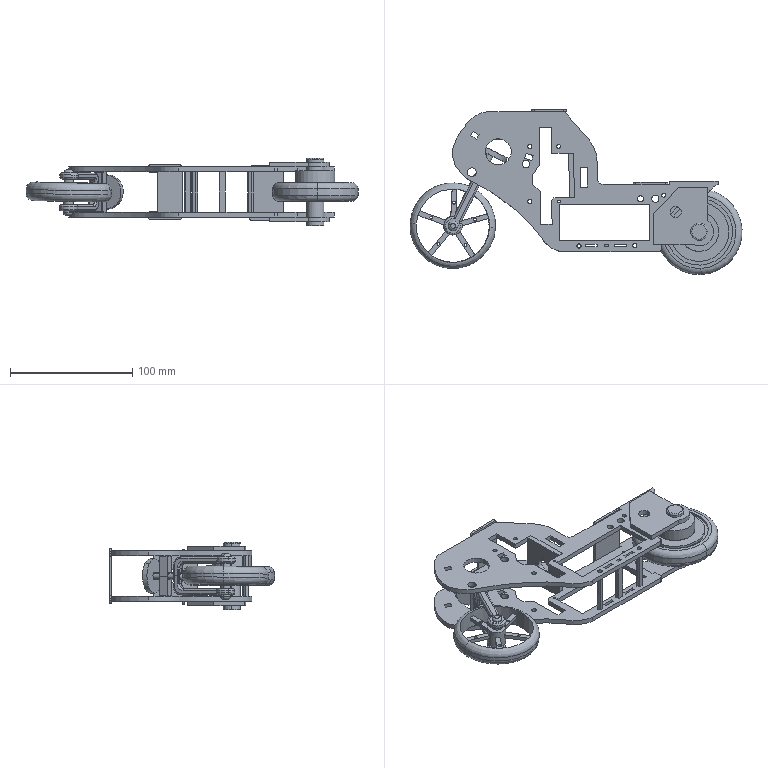Assembly | SolidWorks | mm | 17 component files | 18 solids | 481 faces | box 271.57 x 135.08 x 55 mm | volume 177248 mm3 | plane 239 | cylinder 194 | torus 36 | sphere 8 | spline 4 | commonest cylinder face diameters 2 x16 3 x13 1 x13 8 x10 2.368 x10 4 x10 15 x8 3.467 x8
Bill of materials:
ConnectingBlock1 | 1 |  | Elongated prismatic block, roughly square in cross-section, with lightly rounded edges and a single round cross hole through the side faces.
ConnectingBlock | 1 |  | U-shaped yoke/clevis-like bracket: two parallel arms joined by a rounded base, each arm ending in a flat ring eye with a round hole, and a round hole through the base web.
HexStandoff | 2 |  | Long hollow hexagonal-section tube with a circular bore running the full length; looks like a hex standoff or spacer.
LowerBaffle | 1 |  | Thin flat rectangular plate with rounded corners and four small round holes, one near each corner.
MiddleBaffle | 1 |  | Square flat plate with sharp edges, a large central circular through hole, and four small holes evenly spaced at 90 degrees on a circle around it.
MiddleShortPlate | 1 |  | Plain solid rectangular bar/prism with sharp edges and no holes or other features.
MirrorRearSidePlate1 | 1 |  | Flat plate with one chamfered (angled) corner, a smaller round hole, and a larger round hole set in a rounded lobe that sticks out past one edge.
MirrorSidePlate | 1 |  | Thin flat plate with a complex irregular outline (curved lobe on one end, long narrow tab on the other ending in a concave arc notch) and many cutouts: a large round hole, several small round holes, small rectangular slots, a cross-shaped opening, and a large rectangular window.
Motor | 1 |  | Stepped cylindrical pin with a wider disc-shaped collar near one end, a short cylindrical stub above the collar, and a longer shank of the same diameter below it; ends have small edge rounds.
Part15 | 1 |  | Flat circular disc with a single slender cylindrical pin sticking out perpendicular from the center of one face; pin tip is rounded or chamfered.
RearSidePlate1 | 1 |  | Flat plate with one chamfered (angled) corner, a smaller round hole, and a larger round hole set in a rounded lobe that sticks out past one edge.
RearWheel | 1 |  | Annular disc/ring with a well-rounded outer edge, a central through bore with a larger counterbore step on one face, and a shallow circular groove on that same face.
SidePlate | 1 |  | Thin flat plate with an irregular profile. One end is a rounded lobe and the other is a long narrow arm. The plate has a large round hole, several small round holes, small square/rectangular holes, a large rectangular window, a stepped cross-shaped cutout and a row of small slots.
Tire | 1 |  | Wheel-like ring with five spokes. It has an outer rim with a rounded (toroidal-looking) profile, an open center, and five straight flat spokes running from a cylindrical central hub with a round bore. Each spoke has one small through-hole.
UpperBaffle | 1 |  | Flat rectangular plate with rounded corners. One long side has a wide rectangular recess, which leaves two tabs. There are four small round through-holes, one near each corner, two of them in the tabs.
VehicleRearAxis | 1 |  | Solid round rod or pin with rounded or chamfered ends at both sides. The end view shows a circular cross-section with a slightly domed, faceted end face.
Mates:
1. concentric | Tire-1 face at (-9.114, -6.81, -21.475) dir (0.01984, -0.009985, 0.9998) r 4 | ConnectingBlock-3 face at (-8.36, -7.189, 16.515) dir (-0.01984, 0.009985, -0.9998) r 4
2. concentric | ConnectingBlock-3 face at (-8.36, -7.189, 16.515) dir (-0.01984, 0.009985, -0.9998) r 4 | VehicleRearAxis-1 face at (-8.311, -7.214, 19.015) dir (-0.01984, 0.009985, -0.9998) r 4
3. lock | MirrorSidePlate-2 reference at (0, 0, 0) dir (1, 0, 0) | MiddleBaffle-1 reference at (0, 0, 0) dir (1, 0, 0)
4. concentric | MirrorSidePlate-2 face at (140.23, -23.235, -19.5) dir (0, 0, 1) r 1.733 | HexStandoff-1 face at (140.23, -23.235, 17.5) dir (0, 0, -1) r 1.735
5. coincident | MirrorSidePlate-2 face at (149.645, -1170.52, -15.5) dir (0, 0, 1) | HexStandoff-1 edge at (137.765, -22.777, -15.5) dir (0.6619, 0.7496, 0)
6. concentric | MirrorSidePlate-2 face at (94.514, -23.577, -19.5) dir (0, 0, 1) r 1.733 | HexStandoff-2 face at (94.514, -23.577, 17.5) dir (0, 0, -1) r 1.735
7. coincident | MirrorSidePlate-2 face at (149.645, -1170.52, -15.5) dir (0, 0, 1) | HexStandoff-2 face at (-60.744, 0.3563, -15.5) dir (0, 0, -1)
8. lock | SidePlate-1 reference at (0, 0, 0) dir (1, 0, 0) | MiddleShortPlate-1 reference at (0, 0, 0) dir (1, 0, 0)
9. coincident | MirrorSidePlate-2 face at (154.566, 26.455, -19.5) dir (0.004111, 1, 0) | LowerBaffle-1 face at (64.806, 26.824, -0.2506) dir (-0.004111, -1, 0)
10. lock | SidePlate-1 reference at (0, 0, 0) dir (1, 0, 0) | MirrorSidePlate-2 reference at (0, 0, 0) dir (1, 0, 0)
11. lock | SidePlate-1 reference at (0, 0, 0) dir (1, 0, 0) | RearSidePlate1-1 reference at (0, 0, 0) dir (1, 0, 0)
12. lock | SidePlate-1 reference at (0, 0, 0) dir (1, 0, 0) | LowerBaffle-1 reference at (0, 0, 0) dir (1, 0, 0)
13. width | SidePlate-1 face at (149.645, -1170.52, 17.5) dir (0, 0, -1) | MirrorSidePlate-2 face at (149.645, -1170.52, -15.5) dir (0, 0, 1) | RearWheel-1 face at (192.878, -12.023, 8.5) dir (0, 0, 1) | RearWheel-1 face at (192.878, -12.023, -6.5) dir (0, 0, -1)
14. concentric | RearSidePlate1-1 face at (192.878, -12.023, 25.5) dir (0, 0, -1) r 11.615 | Motor-1 face at (192.878, -12.023, 28.5) dir (0, 0, -1) r 7.09
15. concentric | RearWheel-1 face at (192.878, -12.023, -1.5) dir (0, 0, 1) r 16.004 | Motor-1 face at (192.878, -12.023, 18.5) dir (0, 0, -1) r 16.004
16. distance | Motor-1 face at (192.878, -12.023, 28.5) dir (0, 0, 1) | RearSidePlate1-1 face at (192.878, -12.023, 25.5) dir (0, 0, 1)
17. concentric | ConnectingBlock-3 face at (-12.66, -16.896, 1) dir (0.4496, 0.8932, 0) r 3 | Part15-1 face at (9.872, 27.871, 1) dir (0.4496, 0.8932, 0) r 3
18. lock | SidePlate-1 reference at (0, 0, 0) dir (1, 0, 0) | Part15-1 reference at (0, 0, 0) dir (1, 0, 0)
19. distance | ConnectingBlock-3 face at (14.119, 28.023, 13.42) dir (-0.4496, -0.8932, 0) | Part15-1 face at (9.872, 27.871, 1) dir (-0.4496, -0.8932, 0)
20. concentric | Part15-1 face at (9.872, 27.871, 1) dir (0.4496, 0.8932, 0) r 3 | ConnectingBlock1-1 face at (-12.66, -16.896, 1) dir (0.4496, 0.8932, 0) r 3
21. distance | ConnectingBlock-3 face at (10.214, 35.93, 11.576) dir (0.4496, 0.8932, 0) | ConnectingBlock1-1 face at (14.65, 39.295, 12.5) dir (-0.4496, -0.8932, 0)
22. coincident | MirrorSidePlate-2 face at (149.645, -1170.52, -15.5) dir (0, 0, 1) | ConnectingBlock1-1 face at (15.882, 47.632, -15.5) dir (0, 0, -1)
23. distance | VehicleRearAxis-1 face at (-8.311, -7.214, 19.015) dir (0.01984, -0.009985, 0.9998) | ConnectingBlock-3 face at (-8.36, -7.189, 16.515) dir (0.01984, -0.009985, 0.9998)
24. width | ConnectingBlock-3 face at (-8.876, -6.93, -9.478) dir (0.01984, -0.009985, 0.9998) | ConnectingBlock-3 face at (-8.46, -7.139, 11.517) dir (-0.01984, 0.009985, -0.9998) | Tire-1 face at (-8.817, -6.96, -6.479) dir (-0.01984, 0.009985, -0.9998) | Tire-1 face at (-8.519, -7.109, 8.517) dir (0.01984, -0.009985, 0.9998)
25. lock | SidePlate-1 reference at (0, 0, 0) dir (1, 0, 0) | UpperBaffle-1 reference at (0, 0, 0) dir (1, 0, 0)